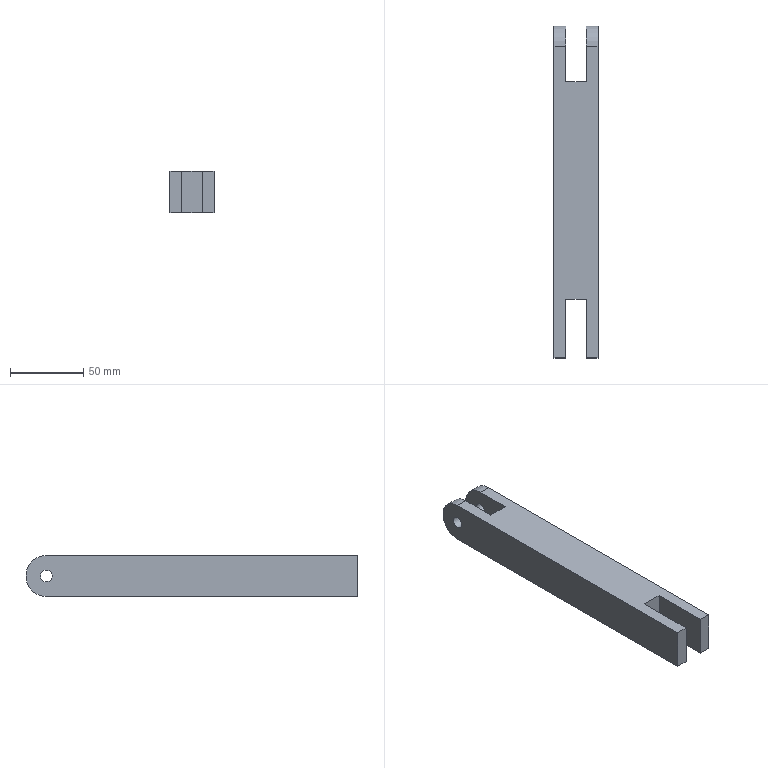Component | NX | CLAMP_PLATE | 1 solid | 16 faces | volume 157114 mm3 | plane 12 | cylinder 4 | commonest cylinder face diameters 28 x2 8 x2